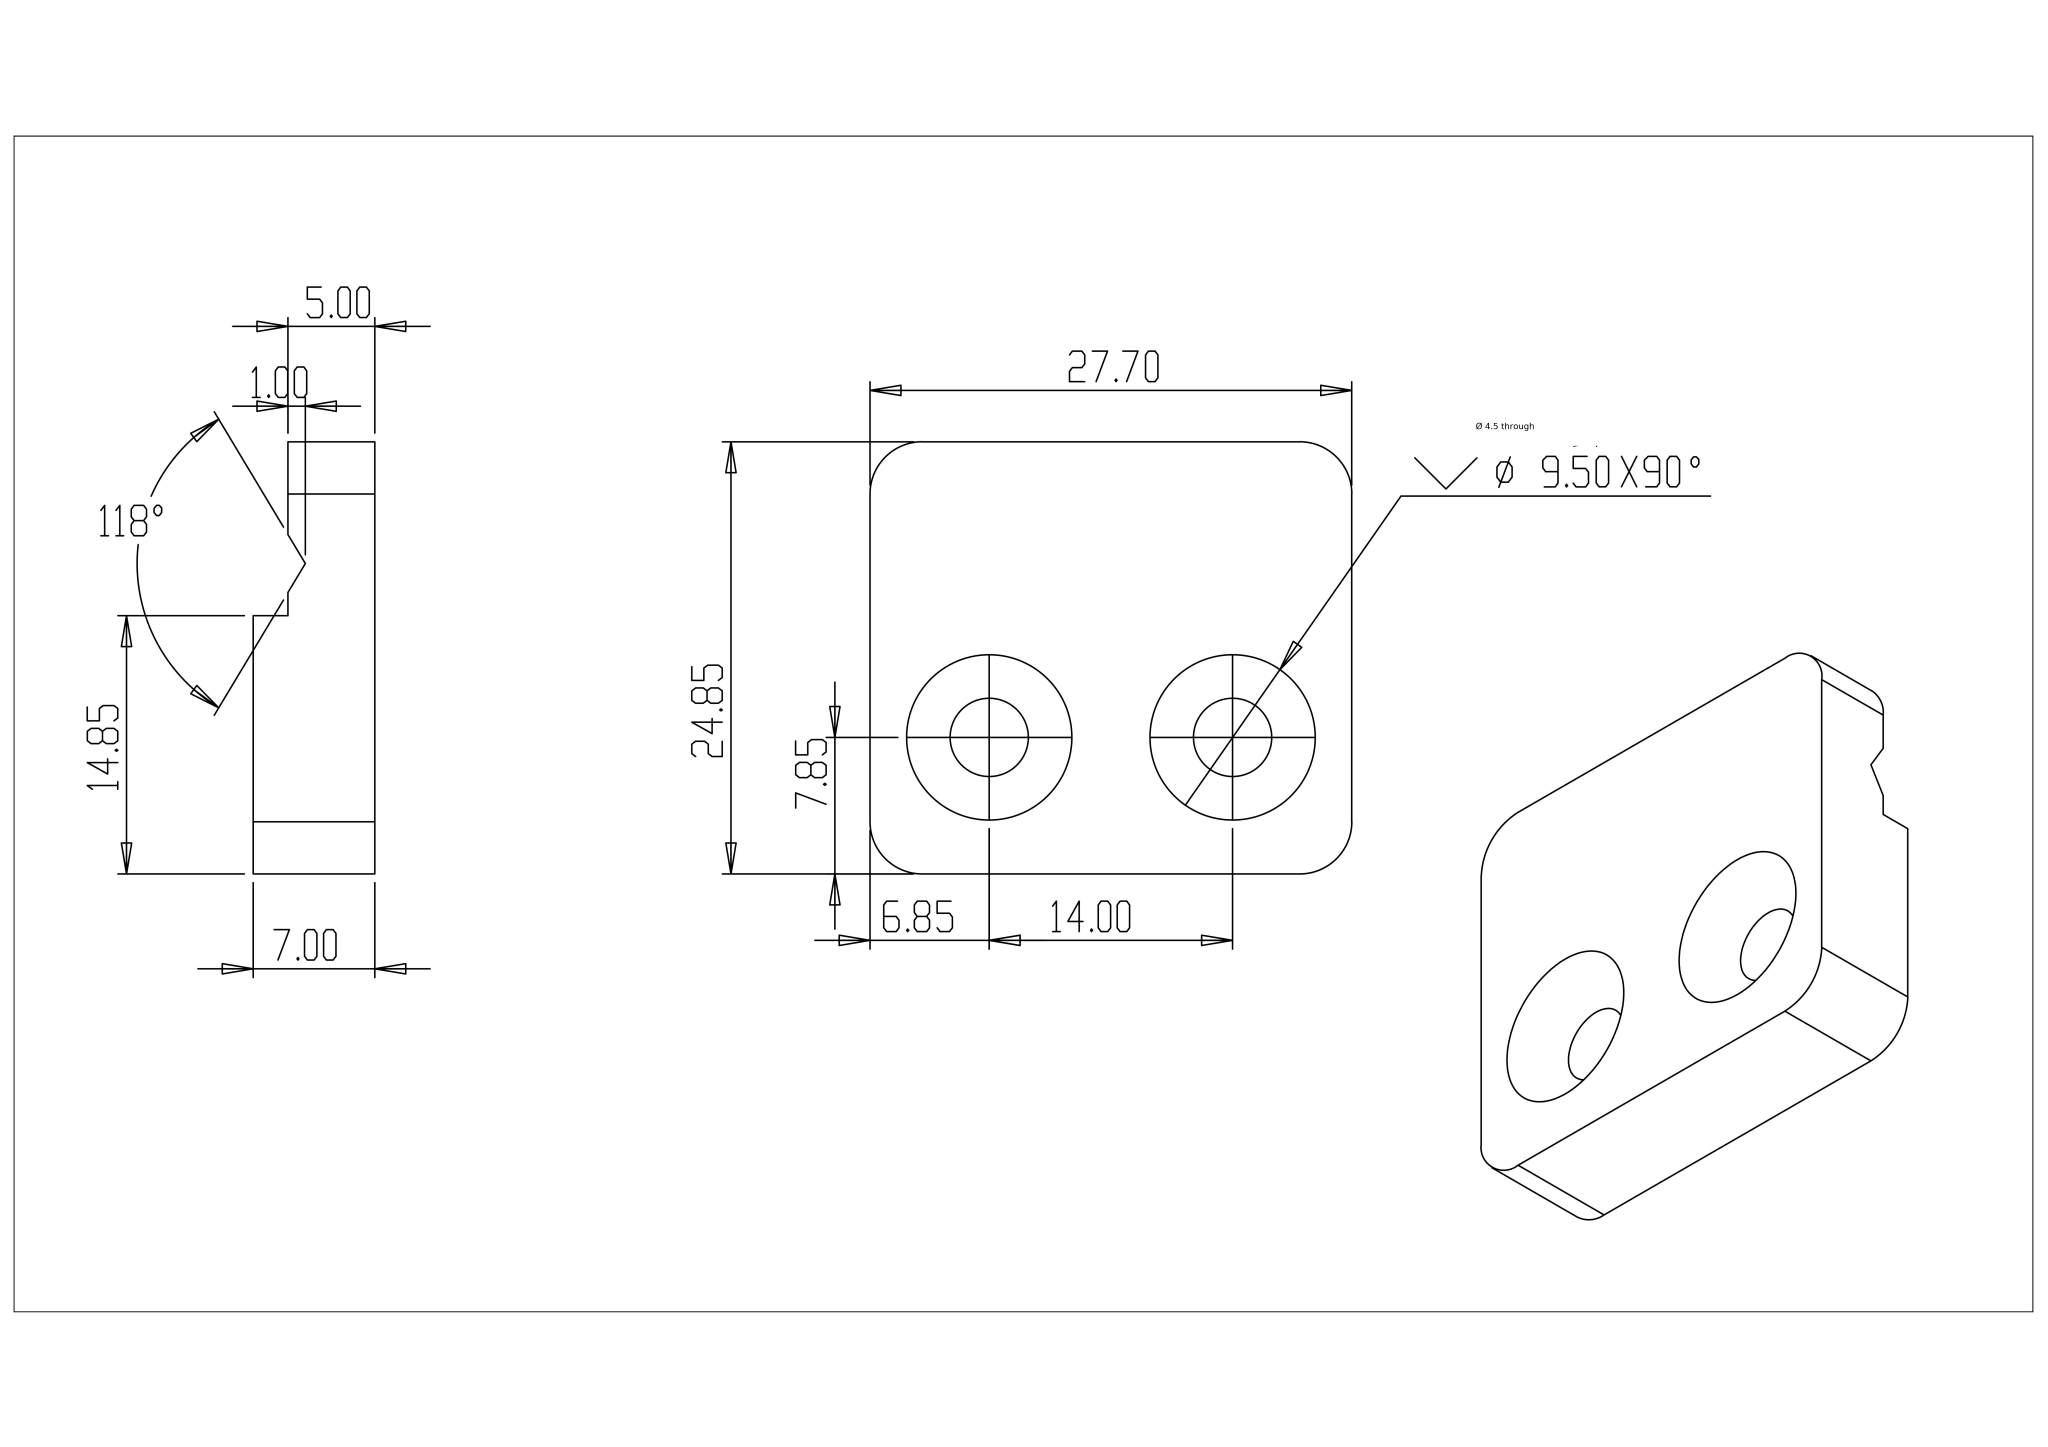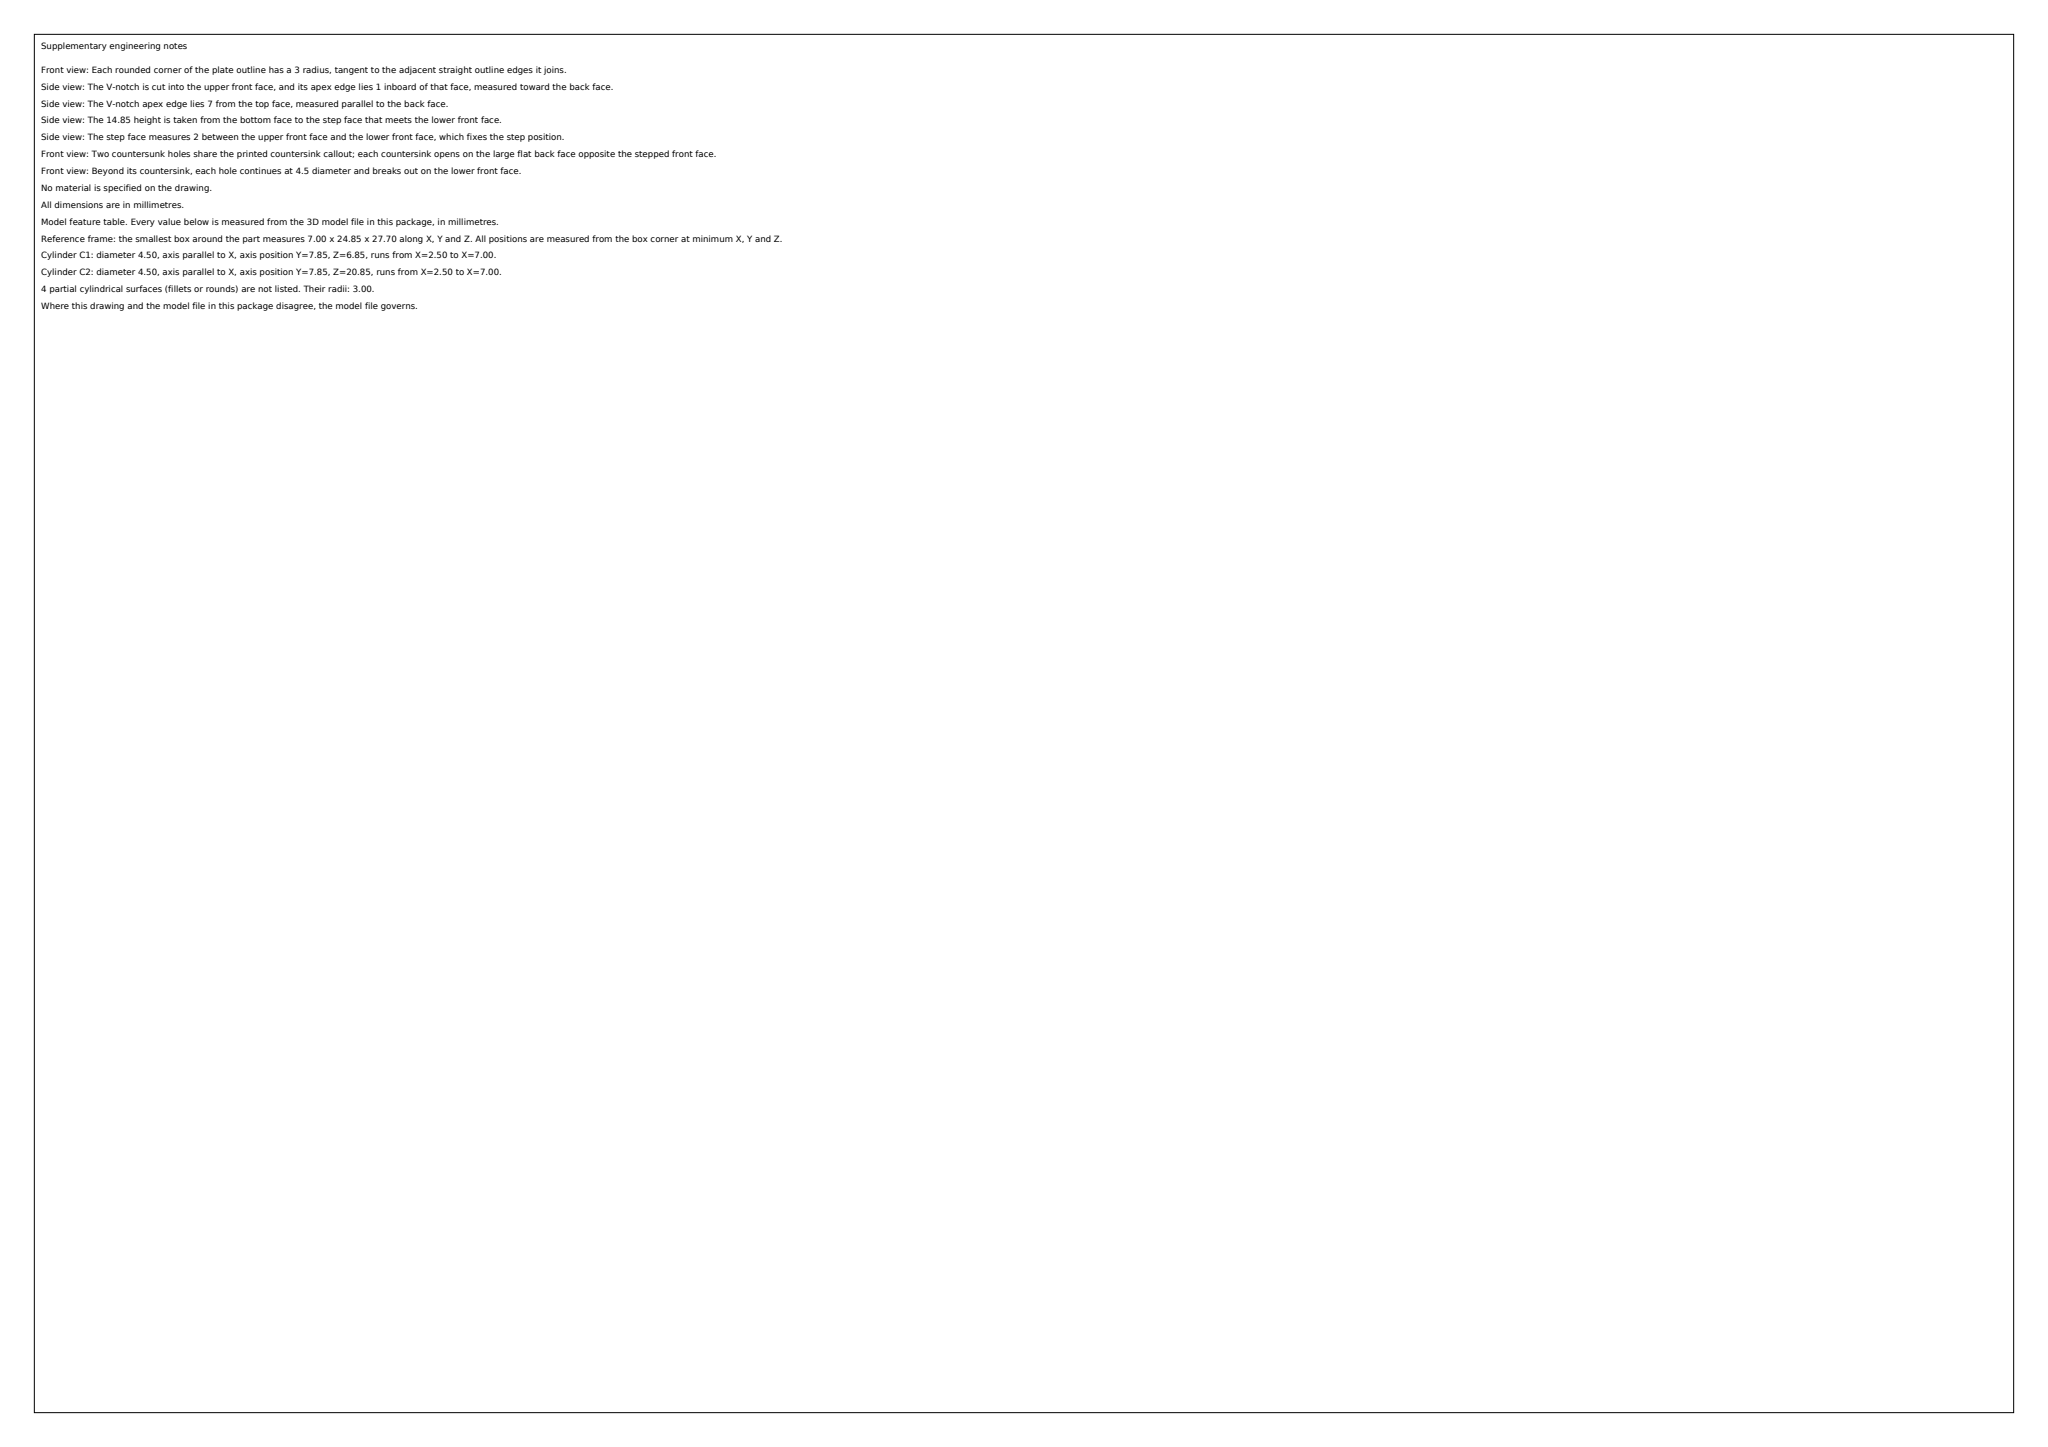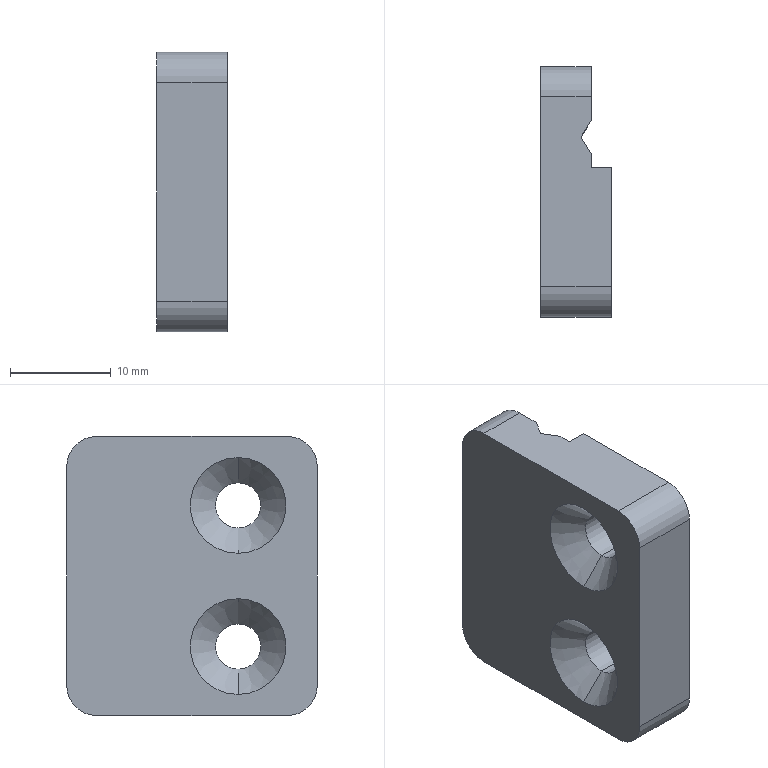Part | SolidWorks | mm | 1 solid | 23 faces | box 7 x 24.85 x 27.7 mm | volume 3828 mm3 | plane 11 | cylinder 8 | cone 4 | commonest cylinder face diameters 4.5 x4 6 x4
Drawing notes:
Ø9.50 X 90° CSK NEAR & FAR SIDE | from the solid: cones[90.0,ref_dia 4.5] count=4 for 2 thru holes -> csk on both x=0 and x=7/5 faces
2X Ø4.5 THRU, CSK Ø9.50 X 90° BOTH SIDES | from the solid: cylinders dia 4.5 at (y7.85,z6.85) and (y7.85,z20.85), 4 cones total
UNLESS OTHERWISE SPECIFIED ALL DIMS IN MM | from the solid: bbox_xyz 7.0 x 24.85 x 27.7 mm
SIDE VIEW: DEL 1.00; BACK STEP 2.00 DP X 10.00 FROM TOP EDGE | from the solid: x planes 0/5/7: 5.0 thk for y 14.85-24.85 (10.00 wide), 7.0 thk below; no face at 1.00
SIDE VIEW: DEL 118°; STEP FACES SQUARE, NO ANGLED FACE | from the solid: axis_planes only normals x,y,z (x=0,5,7; y=0,14.85,24.85; z=0,27.7); no inclined plane
build123d program:
from build123d import *

# Parameters (mm, degrees)
BOSS_EXTRUDE1_DEPTH = 27.7
FILLET1_R           = 3
CUT_EXTRUDE1_REACH  = 39.866
CHAMFER1_SIZE       = 2.5


with BuildPart() as part:
    # Sketch1 → Boss-Extrude1 (new body)
    with BuildSketch(Plane.XY):
        Polygon((0, -22), (0, -24.85), (7, -24.85), (7, -22), (7, -10), (5.3, -10), (5, -10), (5, -8.667), (4, -7), (5, -5.333), (5, -4.5), (5, -3), (5, 0), (0, 0), (0, -3), align=None)
    extrude(amount=BOSS_EXTRUDE1_DEPTH)

    # Fillet1
    fillet1_edges = [part.edges().sort_by_distance(p)[0] for p in [
        (3.5, -24.85, 27.7),
        (2.5, 0, 0),
        (3.5, -24.85, 0),
        (2.5, 0, 27.7),
    ]]
    fillet(fillet1_edges, radius=FILLET1_R)

    # Sketch2 → Cut-Extrude1 (cut, up to next)
    with BuildSketch(Plane(origin=(7, 0, 0), x_dir=(0, 0, -1), z_dir=(1, 0, 0)), mode=Mode.PRIVATE) as cut_extrude1_sk1:
        with BuildLine():
            ThreePointArc((-9.1, -17), (-6.85, -19.25), (-4.6, -17))
            ThreePointArc((-4.6, -17), (-6.85, -14.75), (-9.1, -17))
        make_face()
    cut_extrude1_tool1 = extrude(cut_extrude1_sk1.sketch, amount=-CUT_EXTRUDE1_REACH, mode=Mode.PRIVATE) & part.part
    # Sketch2 → Cut-Extrude1 (cut, up to next)
    with BuildSketch(Plane(origin=(7, 0, 0), x_dir=(0, 0, -1), z_dir=(1, 0, 0)), mode=Mode.PRIVATE) as cut_extrude1_sk2:
        with BuildLine():
            ThreePointArc((-23.1, -17), (-20.85, -19.25), (-18.6, -17))
            ThreePointArc((-18.6, -17), (-20.85, -14.75), (-23.1, -17))
        make_face()
    cut_extrude1_tool2 = extrude(cut_extrude1_sk2.sketch, amount=-CUT_EXTRUDE1_REACH, mode=Mode.PRIVATE) & part.part
    add(cut_extrude1_tool1.solids().sort_by_distance((7, -17, 6.85))[0], mode=Mode.SUBTRACT)
    add(cut_extrude1_tool2.solids().sort_by_distance((7, -17, 20.85))[0], mode=Mode.SUBTRACT)

    # Chamfer1
    chamfer1_edges = [part.edges().sort_by_distance(p)[0] for p in [
        (0, -17, 9.1),
        (0, -17, 18.6),
    ]]
    chamfer(chamfer1_edges, length=CHAMFER1_SIZE)


solid = part.part
STEP:
#1=CARTESIAN_POINT('',(2.5,-17.,4.6));
#2=VERTEX_POINT('',#1);
#3=CARTESIAN_POINT('',(2.5,-17.,9.1));
#4=VERTEX_POINT('',#3);
#5=CARTESIAN_POINT('',(2.5,-17.,6.85));
#6=DIRECTION('',(-1.,0.,0.));
#7=DIRECTION('',(0.,0.,-1.));
#8=AXIS2_PLACEMENT_3D('',#5,#6,#7);
#9=CIRCLE('',#8,2.25);
#10=EDGE_CURVE('',#2,#4,#9,.T.);
#11=ORIENTED_EDGE('',*,*,#10,.F.);
#12=CARTESIAN_POINT('',(0.,-17.,2.1));
#13=VERTEX_POINT('',#12);
#14=CARTESIAN_POINT('',(2.5,-17.,4.6));
#15=DIRECTION('',(-0.7071,0.,-0.7071));
#16=VECTOR('',#15,1000.);
#17=LINE('',#14,#16);
#18=EDGE_CURVE('',#2,#13,#17,.T.);
#19=ORIENTED_EDGE('',*,*,#18,.T.);
#20=CARTESIAN_POINT('',(0.,-17.,11.6));
#21=VERTEX_POINT('',#20);
#22=CARTESIAN_POINT('',(0.,-17.,6.85));
#23=DIRECTION('',(1.,0.,0.));
#24=DIRECTION('',(0.,0.,-1.));
#25=AXIS2_PLACEMENT_3D('',#22,#23,#24);
#26=CIRCLE('',#25,4.75);
#27=EDGE_CURVE('',#21,#13,#26,.T.);
#28=ORIENTED_EDGE('',*,*,#27,.F.);
#29=CARTESIAN_POINT('',(2.5,-17.,9.1));
#30=DIRECTION('',(-0.7071,0.,0.7071));
#31=VECTOR('',#30,1000.);
#32=LINE('',#29,#31);
#33=EDGE_CURVE('',#4,#21,#32,.T.);
#34=ORIENTED_EDGE('',*,*,#33,.F.);
#35=EDGE_LOOP('',(#11,#19,#28,#34));
#36=FACE_OUTER_BOUND('',#35,.T.);
#37=CARTESIAN_POINT('',(2.5,-17.,6.85));
#38=DIRECTION('',(-1.,0.,0.));
#39=DIRECTION('',(0.,0.,1.));
#40=AXIS2_PLACEMENT_3D('',#37,#38,#39);
#41=CONICAL_SURFACE('',#40,2.25,0.7854);
#42=ADVANCED_FACE('',(#36),#41,.F.);
#43=CARTESIAN_POINT('',(2.5,-17.,18.6));
#44=VERTEX_POINT('',#43);
#45=CARTESIAN_POINT('',(2.5,-17.,23.1));
#46=VERTEX_POINT('',#45);
#47=CARTESIAN_POINT('',(2.5,-17.,20.85));
#48=DIRECTION('',(-1.,0.,0.));
#49=DIRECTION('',(0.,0.,-1.));
#50=AXIS2_PLACEMENT_3D('',#47,#48,#49);
#51=CIRCLE('',#50,2.25);
#52=EDGE_CURVE('',#44,#46,#51,.T.);
#53=ORIENTED_EDGE('',*,*,#52,.F.);
#54=CARTESIAN_POINT('',(0.,-17.,16.1));
#55=VERTEX_POINT('',#54);
#56=CARTESIAN_POINT('',(2.5,-17.,18.6));
#57=DIRECTION('',(-0.7071,0.,-0.7071));
#58=VECTOR('',#57,1000.);
#59=LINE('',#56,#58);
#60=EDGE_CURVE('',#44,#55,#59,.T.);
#61=ORIENTED_EDGE('',*,*,#60,.T.);
#62=CARTESIAN_POINT('',(0.,-17.,25.6));
#63=VERTEX_POINT('',#62);
#64=CARTESIAN_POINT('',(0.,-17.,20.85));
#65=DIRECTION('',(1.,0.,0.));
#66=DIRECTION('',(0.,0.,-1.));
#67=AXIS2_PLACEMENT_3D('',#64,#65,#66);
#68=CIRCLE('',#67,4.75);
#69=EDGE_CURVE('',#63,#55,#68,.T.);
#70=ORIENTED_EDGE('',*,*,#69,.F.);
#71=CARTESIAN_POINT('',(2.5,-17.,23.1));
#72=DIRECTION('',(-0.7071,0.,0.7071));
#73=VECTOR('',#72,1000.);
#74=LINE('',#71,#73);
#75=EDGE_CURVE('',#46,#63,#74,.T.);
#76=ORIENTED_EDGE('',*,*,#75,.F.);
#77=EDGE_LOOP('',(#53,#61,#70,#76));
#78=FACE_OUTER_BOUND('',#77,.T.);
#79=CARTESIAN_POINT('',(2.5,-17.,20.85));
#80=DIRECTION('',(-1.,0.,0.));
#81=DIRECTION('',(0.,0.,1.));
#82=AXIS2_PLACEMENT_3D('',#79,#80,#81);
#83=CONICAL_SURFACE('',#82,2.25,0.7854);
#84=ADVANCED_FACE('',(#78),#83,.F.);
#85=ORIENTED_EDGE('',*,*,#10,.T.);
#86=CARTESIAN_POINT('',(7.,-17.,9.1));
#87=VERTEX_POINT('',#86);
#88=CARTESIAN_POINT('',(-0.001,-17.,9.1));
#89=DIRECTION('',(1.,0.,0.));
#90=VECTOR('',#89,1000.);
#91=LINE('',#88,#90);
#92=EDGE_CURVE('',#4,#87,#91,.T.);
#93=ORIENTED_EDGE('',*,*,#92,.T.);
#94=CARTESIAN_POINT('',(7.,-17.,4.6));
#95=VERTEX_POINT('',#94);
#96=CARTESIAN_POINT('',(7.,-17.,6.85));
#97=DIRECTION('',(1.,0.,0.));
#98=DIRECTION('',(0.,0.,-1.));
#99=AXIS2_PLACEMENT_3D('',#96,#97,#98);
#100=CIRCLE('',#99,2.25);
#101=EDGE_CURVE('',#87,#95,#100,.T.);
#102=ORIENTED_EDGE('',*,*,#101,.T.);
#103=CARTESIAN_POINT('',(-0.001,-17.,4.6));
#104=DIRECTION('',(1.,0.,0.));
#105=VECTOR('',#104,1000.);
#106=LINE('',#103,#105);
#107=EDGE_CURVE('',#2,#95,#106,.T.);
#108=ORIENTED_EDGE('',*,*,#107,.F.);
#109=EDGE_LOOP('',(#85,#93,#102,#108));
#110=FACE_OUTER_BOUND('',#109,.T.);
#111=CARTESIAN_POINT('',(-0.001,-17.,6.85));
#112=DIRECTION('',(1.,0.,0.));
#113=DIRECTION('',(0.,0.,-1.));
#114=AXIS2_PLACEMENT_3D('',#111,#112,#113);
#115=CYLINDRICAL_SURFACE('',#114,2.25);
#116=ADVANCED_FACE('',(#110),#115,.F.);
#117=ORIENTED_EDGE('',*,*,#52,.T.);
#118=CARTESIAN_POINT('',(7.,-17.,23.1));
#119=VERTEX_POINT('',#118);
#120=CARTESIAN_POINT('',(-0.001,-17.,23.1));
#121=DIRECTION('',(1.,0.,0.));
#122=VECTOR('',#121,1000.);
#123=LINE('',#120,#122);
#124=EDGE_CURVE('',#46,#119,#123,.T.);
#125=ORIENTED_EDGE('',*,*,#124,.T.);
#126=CARTESIAN_POINT('',(7.,-17.,18.6));
#127=VERTEX_POINT('',#126);
#128=CARTESIAN_POINT('',(7.,-17.,20.85));
#129=DIRECTION('',(1.,0.,0.));
#130=DIRECTION('',(0.,0.,-1.));
#131=AXIS2_PLACEMENT_3D('',#128,#129,#130);
#132=CIRCLE('',#131,2.25);
#133=EDGE_CURVE('',#119,#127,#132,.T.);
#134=ORIENTED_EDGE('',*,*,#133,.T.);
#135=CARTESIAN_POINT('',(-0.001,-17.,18.6));
#136=DIRECTION('',(1.,0.,0.));
#137=VECTOR('',#136,1000.);
#138=LINE('',#135,#137);
#139=EDGE_CURVE('',#44,#127,#138,.T.);
#140=ORIENTED_EDGE('',*,*,#139,.F.);
#141=EDGE_LOOP('',(#117,#125,#134,#140));
#142=FACE_OUTER_BOUND('',#141,.T.);
#143=CARTESIAN_POINT('',(-0.001,-17.,20.85));
#144=DIRECTION('',(1.,0.,0.));
#145=DIRECTION('',(0.,0.,-1.));
#146=AXIS2_PLACEMENT_3D('',#143,#144,#145);
#147=CYLINDRICAL_SURFACE('',#146,2.25);
#148=ADVANCED_FACE('',(#142),#147,.F.);
#149=CARTESIAN_POINT('',(0.,-24.85,24.7));
#150=VERTEX_POINT('',#149);
#151=CARTESIAN_POINT('',(0.,-24.85,3.));
#152=VERTEX_POINT('',#151);
#153=CARTESIAN_POINT('',(0.,-24.85,27.7));
#154=DIRECTION('',(0.,0.,-1.));
#155=VECTOR('',#154,1000.);
#156=LINE('',#153,#155);
#157=EDGE_CURVE('',#150,#152,#156,.T.);
#158=ORIENTED_EDGE('',*,*,#157,.T.);
#159=CARTESIAN_POINT('',(7.,-24.85,3.));
#160=VERTEX_POINT('',#159);
#161=CARTESIAN_POINT('',(0.,-24.85,3.));
#162=DIRECTION('',(1.,0.,0.));
#163=VECTOR('',#162,1000.);
#164=LINE('',#161,#163);
#165=EDGE_CURVE('',#152,#160,#164,.T.);
#166=ORIENTED_EDGE('',*,*,#165,.T.);
#167=CARTESIAN_POINT('',(7.,-24.85,24.7));
#168=VERTEX_POINT('',#167);
#169=CARTESIAN_POINT('',(7.,-24.85,27.7));
#170=DIRECTION('',(0.,0.,-1.));
#171=VECTOR('',#170,1000.);
#172=LINE('',#169,#171);
#173=EDGE_CURVE('',#168,#160,#172,.T.);
#174=ORIENTED_EDGE('',*,*,#173,.F.);
#175=CARTESIAN_POINT('',(0.,-24.85,24.7));
#176=DIRECTION('',(-1.,0.,0.));
#177=VECTOR('',#176,1000.);
#178=LINE('',#175,#177);
#179=EDGE_CURVE('',#168,#150,#178,.T.);
#180=ORIENTED_EDGE('',*,*,#179,.T.);
#181=EDGE_LOOP('',(#158,#166,#174,#180));
#182=FACE_OUTER_BOUND('',#181,.T.);
#183=CARTESIAN_POINT('',(0.,-24.85,27.7));
#184=DIRECTION('',(0.,1.,0.));
#185=DIRECTION('',(0.,0.,1.));
#186=AXIS2_PLACEMENT_3D('',#183,#184,#185);
#187=PLANE('',#186);
#188=ADVANCED_FACE('',(#182),#187,.F.);
#189=CARTESIAN_POINT('',(7.,-17.,6.85));
#190=DIRECTION('',(1.,0.,0.));
#191=DIRECTION('',(0.,0.,-1.));
#192=AXIS2_PLACEMENT_3D('',#189,#190,#191);
#193=CIRCLE('',#192,2.25);
#194=EDGE_CURVE('',#95,#87,#193,.T.);
#195=ORIENTED_EDGE('',*,*,#194,.F.);
#196=ORIENTED_EDGE('',*,*,#101,.F.);
#197=EDGE_LOOP('',(#195,#196));
#198=FACE_BOUND('',#197,.T.);
#199=CARTESIAN_POINT('',(7.,-17.,20.85));
#200=DIRECTION('',(1.,0.,0.));
#201=DIRECTION('',(0.,0.,-1.));
#202=AXIS2_PLACEMENT_3D('',#199,#200,#201);
#203=CIRCLE('',#202,2.25);
#204=EDGE_CURVE('',#127,#119,#203,.T.);
#205=ORIENTED_EDGE('',*,*,#204,.F.);
#206=ORIENTED_EDGE('',*,*,#133,.F.);
#207=EDGE_LOOP('',(#205,#206));
#208=FACE_BOUND('',#207,.T.);
#209=ORIENTED_EDGE('',*,*,#173,.T.);
#210=CARTESIAN_POINT('',(7.,-21.85,0.));
#211=VERTEX_POINT('',#210);
#212=CARTESIAN_POINT('',(7.,-21.85,3.));
#213=DIRECTION('',(1.,0.,0.));
#214=DIRECTION('',(0.,0.,1.));
#215=AXIS2_PLACEMENT_3D('',#212,#213,#214);
#216=CIRCLE('',#215,3.);
#217=EDGE_CURVE('',#160,#211,#216,.T.);
#218=ORIENTED_EDGE('',*,*,#217,.T.);
#219=CARTESIAN_POINT('',(7.,-10.,0.));
#220=VERTEX_POINT('',#219);
#221=CARTESIAN_POINT('',(7.,-22.,0.));
#222=DIRECTION('',(0.,1.,0.));
#223=VECTOR('',#222,1000.);
#224=LINE('',#221,#223);
#225=EDGE_CURVE('',#211,#220,#224,.T.);
#226=ORIENTED_EDGE('',*,*,#225,.T.);
#227=CARTESIAN_POINT('',(7.,-10.,27.7));
#228=VERTEX_POINT('',#227);
#229=CARTESIAN_POINT('',(7.,-10.,27.7));
#230=DIRECTION('',(0.,0.,-1.));
#231=VECTOR('',#230,1000.);
#232=LINE('',#229,#231);
#233=EDGE_CURVE('',#228,#220,#232,.T.);
#234=ORIENTED_EDGE('',*,*,#233,.F.);
#235=CARTESIAN_POINT('',(7.,-21.85,27.7));
#236=VERTEX_POINT('',#235);
#237=CARTESIAN_POINT('',(7.,-24.85,27.7));
#238=DIRECTION('',(0.,1.,0.));
#239=VECTOR('',#238,1000.);
#240=LINE('',#237,#239);
#241=EDGE_CURVE('',#236,#228,#240,.T.);
#242=ORIENTED_EDGE('',*,*,#241,.F.);
#243=CARTESIAN_POINT('',(7.,-21.85,24.7));
#244=DIRECTION('',(1.,0.,0.));
#245=DIRECTION('',(0.,0.,1.));
#246=AXIS2_PLACEMENT_3D('',#243,#244,#245);
#247=CIRCLE('',#246,3.);
#248=EDGE_CURVE('',#236,#168,#247,.T.);
#249=ORIENTED_EDGE('',*,*,#248,.T.);
#250=EDGE_LOOP('',(#209,#218,#226,#234,#242,#249));
#251=FACE_OUTER_BOUND('',#250,.T.);
#252=CARTESIAN_POINT('',(7.,-22.,27.7));
#253=DIRECTION('',(-1.,0.,0.));
#254=DIRECTION('',(0.,0.,1.));
#255=AXIS2_PLACEMENT_3D('',#252,#253,#254);
#256=PLANE('',#255);
#257=ADVANCED_FACE('',(#198,#208,#251),#256,.F.);
#258=CARTESIAN_POINT('',(5.,-10.,0.));
#259=VERTEX_POINT('',#258);
#260=CARTESIAN_POINT('',(5.,-10.,0.));
#261=DIRECTION('',(-1.,0.,0.));
#262=VECTOR('',#261,1000.);
#263=LINE('',#260,#262);
#264=EDGE_CURVE('',#220,#259,#263,.T.);
#265=ORIENTED_EDGE('',*,*,#264,.T.);
#266=CARTESIAN_POINT('',(5.,-10.,27.7));
#267=VERTEX_POINT('',#266);
#268=CARTESIAN_POINT('',(5.,-10.,27.7));
#269=DIRECTION('',(0.,0.,-1.));
#270=VECTOR('',#269,1000.);
#271=LINE('',#268,#270);
#272=EDGE_CURVE('',#267,#259,#271,.T.);
#273=ORIENTED_EDGE('',*,*,#272,.F.);
#274=CARTESIAN_POINT('',(7.,-10.,27.7));
#275=DIRECTION('',(-1.,0.,0.));
#276=VECTOR('',#275,1000.);
#277=LINE('',#274,#276);
#278=EDGE_CURVE('',#228,#267,#277,.T.);
#279=ORIENTED_EDGE('',*,*,#278,.F.);
#280=ORIENTED_EDGE('',*,*,#233,.T.);
#281=EDGE_LOOP('',(#265,#273,#279,#280));
#282=FACE_OUTER_BOUND('',#281,.T.);
#283=CARTESIAN_POINT('',(5.,-10.,27.7));
#284=DIRECTION('',(0.,-1.,0.));
#285=DIRECTION('',(0.,0.,-1.));
#286=AXIS2_PLACEMENT_3D('',#283,#284,#285);
#287=PLANE('',#286);
#288=ADVANCED_FACE('',(#282),#287,.F.);
#289=CARTESIAN_POINT('',(5.,-8.667,0.));
#290=VERTEX_POINT('',#289);
#291=CARTESIAN_POINT('',(5.,-8.667,0.));
#292=DIRECTION('',(0.,1.,0.));
#293=VECTOR('',#292,1000.);
#294=LINE('',#291,#293);
#295=EDGE_CURVE('',#259,#290,#294,.T.);
#296=ORIENTED_EDGE('',*,*,#295,.T.);
#297=CARTESIAN_POINT('',(5.,-8.667,27.7));
#298=VERTEX_POINT('',#297);
#299=CARTESIAN_POINT('',(5.,-8.667,27.7));
#300=DIRECTION('',(0.,0.,-1.));
#301=VECTOR('',#300,1000.);
#302=LINE('',#299,#301);
#303=EDGE_CURVE('',#298,#290,#302,.T.);
#304=ORIENTED_EDGE('',*,*,#303,.F.);
#305=CARTESIAN_POINT('',(5.,-8.667,27.7));
#306=DIRECTION('',(0.,1.,0.));
#307=VECTOR('',#306,1000.);
#308=LINE('',#305,#307);
#309=EDGE_CURVE('',#267,#298,#308,.T.);
#310=ORIENTED_EDGE('',*,*,#309,.F.);
#311=ORIENTED_EDGE('',*,*,#272,.T.);
#312=EDGE_LOOP('',(#296,#304,#310,#311));
#313=FACE_OUTER_BOUND('',#312,.T.);
#314=CARTESIAN_POINT('',(5.,-8.667,27.7));
#315=DIRECTION('',(-1.,0.,0.));
#316=DIRECTION('',(-0.,-1.,0.));
#317=AXIS2_PLACEMENT_3D('',#314,#315,#316);
#318=PLANE('',#317);
#319=ADVANCED_FACE('',(#313),#318,.F.);
#320=CARTESIAN_POINT('',(4.,-7.,0.));
#321=VERTEX_POINT('',#320);
#322=CARTESIAN_POINT('',(5.,-8.667,0.));
#323=DIRECTION('',(-0.5145,0.8575,0.));
#324=VECTOR('',#323,1000.);
#325=LINE('',#322,#324);
#326=EDGE_CURVE('',#290,#321,#325,.T.);
#327=ORIENTED_EDGE('',*,*,#326,.T.);
#328=CARTESIAN_POINT('',(4.,-7.,27.7));
#329=VERTEX_POINT('',#328);
#330=CARTESIAN_POINT('',(4.,-7.,27.7));
#331=DIRECTION('',(0.,0.,-1.));
#332=VECTOR('',#331,1000.);
#333=LINE('',#330,#332);
#334=EDGE_CURVE('',#329,#321,#333,.T.);
#335=ORIENTED_EDGE('',*,*,#334,.F.);
#336=CARTESIAN_POINT('',(5.,-8.667,27.7));
#337=DIRECTION('',(-0.5145,0.8575,0.));
#338=VECTOR('',#337,1000.);
#339=LINE('',#336,#338);
#340=EDGE_CURVE('',#298,#329,#339,.T.);
#341=ORIENTED_EDGE('',*,*,#340,.F.);
#342=ORIENTED_EDGE('',*,*,#303,.T.);
#343=EDGE_LOOP('',(#327,#335,#341,#342));
#344=FACE_OUTER_BOUND('',#343,.T.);
#345=CARTESIAN_POINT('',(5.,-8.667,27.7));
#346=DIRECTION('',(-0.8575,-0.5145,0.));
#347=DIRECTION('',(0.5145,-0.8575,0.));
#348=AXIS2_PLACEMENT_3D('',#345,#346,#347);
#349=PLANE('',#348);
#350=ADVANCED_FACE('',(#344),#349,.F.);
#351=CARTESIAN_POINT('',(5.,-5.333,0.));
#352=VERTEX_POINT('',#351);
#353=CARTESIAN_POINT('',(4.,-7.,0.));
#354=DIRECTION('',(0.5145,0.8575,0.));
#355=VECTOR('',#354,1000.);
#356=LINE('',#353,#355);
#357=EDGE_CURVE('',#321,#352,#356,.T.);
#358=ORIENTED_EDGE('',*,*,#357,.T.);
#359=CARTESIAN_POINT('',(5.,-5.333,27.7));
#360=VERTEX_POINT('',#359);
#361=CARTESIAN_POINT('',(5.,-5.333,27.7));
#362=DIRECTION('',(0.,0.,-1.));
#363=VECTOR('',#362,1000.);
#364=LINE('',#361,#363);
#365=EDGE_CURVE('',#360,#352,#364,.T.);
#366=ORIENTED_EDGE('',*,*,#365,.F.);
#367=CARTESIAN_POINT('',(4.,-7.,27.7));
#368=DIRECTION('',(0.5145,0.8575,0.));
#369=VECTOR('',#368,1000.);
#370=LINE('',#367,#369);
#371=EDGE_CURVE('',#329,#360,#370,.T.);
#372=ORIENTED_EDGE('',*,*,#371,.F.);
#373=ORIENTED_EDGE('',*,*,#334,.T.);
#374=EDGE_LOOP('',(#358,#366,#372,#373));
#375=FACE_OUTER_BOUND('',#374,.T.);
#376=CARTESIAN_POINT('',(4.,-7.,27.7));
#377=DIRECTION('',(-0.8575,0.5145,0.));
#378=DIRECTION('',(-0.5145,-0.8575,0.));
#379=AXIS2_PLACEMENT_3D('',#376,#377,#378);
#380=PLANE('',#379);
#381=ADVANCED_FACE('',(#375),#380,.F.);
#382=CARTESIAN_POINT('',(5.,-3.,0.));
#383=VERTEX_POINT('',#382);
#384=CARTESIAN_POINT('',(5.,-3.,0.));
#385=DIRECTION('',(0.,1.,0.));
#386=VECTOR('',#385,1000.);
#387=LINE('',#384,#386);
#388=EDGE_CURVE('',#352,#383,#387,.T.);
#389=ORIENTED_EDGE('',*,*,#388,.T.);
#390=CARTESIAN_POINT('',(5.,0.,3.));
#391=VERTEX_POINT('',#390);
#392=CARTESIAN_POINT('',(5.,-3.,3.));
#393=DIRECTION('',(1.,0.,0.));
#394=DIRECTION('',(0.,0.,1.));
#395=AXIS2_PLACEMENT_3D('',#392,#393,#394);
#396=CIRCLE('',#395,3.);
#397=EDGE_CURVE('',#383,#391,#396,.T.);
#398=ORIENTED_EDGE('',*,*,#397,.T.);
#399=CARTESIAN_POINT('',(5.,0.,24.7));
#400=VERTEX_POINT('',#399);
#401=CARTESIAN_POINT('',(5.,0.,27.7));
#402=DIRECTION('',(0.,0.,-1.));
#403=VECTOR('',#402,1000.);
#404=LINE('',#401,#403);
#405=EDGE_CURVE('',#400,#391,#404,.T.);
#406=ORIENTED_EDGE('',*,*,#405,.F.);
#407=CARTESIAN_POINT('',(5.,-3.,27.7));
#408=VERTEX_POINT('',#407);
#409=CARTESIAN_POINT('',(5.,-3.,24.7));
#410=DIRECTION('',(1.,0.,0.));
#411=DIRECTION('',(0.,0.,1.));
#412=AXIS2_PLACEMENT_3D('',#409,#410,#411);
#413=CIRCLE('',#412,3.);
#414=EDGE_CURVE('',#400,#408,#413,.T.);
#415=ORIENTED_EDGE('',*,*,#414,.T.);
#416=CARTESIAN_POINT('',(5.,-4.5,27.7));
#417=DIRECTION('',(0.,1.,0.));
#418=VECTOR('',#417,1000.);
#419=LINE('',#416,#418);
#420=EDGE_CURVE('',#360,#408,#419,.T.);
#421=ORIENTED_EDGE('',*,*,#420,.F.);
#422=ORIENTED_EDGE('',*,*,#365,.T.);
#423=EDGE_LOOP('',(#389,#398,#406,#415,#421,#422));
#424=FACE_OUTER_BOUND('',#423,.T.);
#425=CARTESIAN_POINT('',(5.,-3.,27.7));
#426=DIRECTION('',(-1.,0.,0.));
#427=DIRECTION('',(0.,0.,1.));
#428=AXIS2_PLACEMENT_3D('',#425,#426,#427);
#429=PLANE('',#428);
#430=ADVANCED_FACE('',(#424),#429,.F.);
#431=ORIENTED_EDGE('',*,*,#405,.T.);
#432=CARTESIAN_POINT('',(0.,0.,3.));
#433=VERTEX_POINT('',#432);
#434=CARTESIAN_POINT('',(5.,0.,3.));
#435=DIRECTION('',(-1.,0.,0.));
#436=VECTOR('',#435,1000.);
#437=LINE('',#434,#436);
#438=EDGE_CURVE('',#391,#433,#437,.T.);
#439=ORIENTED_EDGE('',*,*,#438,.T.);
#440=CARTESIAN_POINT('',(0.,0.,24.7));
#441=VERTEX_POINT('',#440);
#442=CARTESIAN_POINT('',(0.,0.,27.7));
#443=DIRECTION('',(0.,0.,-1.));
#444=VECTOR('',#443,1000.);
#445=LINE('',#442,#444);
#446=EDGE_CURVE('',#441,#433,#445,.T.);
#447=ORIENTED_EDGE('',*,*,#446,.F.);
#448=CARTESIAN_POINT('',(5.,0.,24.7));
#449=DIRECTION('',(1.,0.,0.));
#450=VECTOR('',#449,1000.);
#451=LINE('',#448,#450);
#452=EDGE_CURVE('',#441,#400,#451,.T.);
#453=ORIENTED_EDGE('',*,*,#452,.T.);
#454=EDGE_LOOP('',(#431,#439,#447,#453));
#455=FACE_OUTER_BOUND('',#454,.T.);
#456=CARTESIAN_POINT('',(5.,0.,27.7));
#457=DIRECTION('',(0.,-1.,0.));
#458=DIRECTION('',(0.,0.,-1.));
#459=AXIS2_PLACEMENT_3D('',#456,#457,#458);
#460=PLANE('',#459);
#461=ADVANCED_FACE('',(#455),#460,.F.);
#462=ORIENTED_EDGE('',*,*,#69,.T.);
#463=CARTESIAN_POINT('',(0.,-17.,20.85));
#464=DIRECTION('',(1.,0.,0.));
#465=DIRECTION('',(0.,0.,-1.));
#466=AXIS2_PLACEMENT_3D('',#463,#464,#465);
#467=CIRCLE('',#466,4.75);
#468=EDGE_CURVE('',#55,#63,#467,.T.);
#469=ORIENTED_EDGE('',*,*,#468,.T.);
#470=EDGE_LOOP('',(#462,#469));
#471=FACE_BOUND('',#470,.T.);
#472=ORIENTED_EDGE('',*,*,#27,.T.);
#473=CARTESIAN_POINT('',(0.,-17.,6.85));
#474=DIRECTION('',(1.,0.,0.));
#475=DIRECTION('',(0.,0.,-1.));
#476=AXIS2_PLACEMENT_3D('',#473,#474,#475);
#477=CIRCLE('',#476,4.75);
#478=EDGE_CURVE('',#13,#21,#477,.T.);
#479=ORIENTED_EDGE('',*,*,#478,.T.);
#480=EDGE_LOOP('',(#472,#479));
#481=FACE_BOUND('',#480,.T.);
#482=ORIENTED_EDGE('',*,*,#446,.T.);
#483=CARTESIAN_POINT('',(0.,-3.,0.));
#484=VERTEX_POINT('',#483);
#485=CARTESIAN_POINT('',(0.,-3.,3.));
#486=DIRECTION('',(-1.,0.,0.));
#487=DIRECTION('',(0.,0.,-1.));
#488=AXIS2_PLACEMENT_3D('',#485,#486,#487);
#489=CIRCLE('',#488,3.);
#490=EDGE_CURVE('',#433,#484,#489,.T.);
#491=ORIENTED_EDGE('',*,*,#490,.T.);
#492=CARTESIAN_POINT('',(0.,-21.85,0.));
#493=VERTEX_POINT('',#492);
#494=CARTESIAN_POINT('',(0.,0.,0.));
#495=DIRECTION('',(0.,-1.,0.));
#496=VECTOR('',#495,1000.);
#497=LINE('',#494,#496);
#498=EDGE_CURVE('',#484,#493,#497,.T.);
#499=ORIENTED_EDGE('',*,*,#498,.T.);
#500=CARTESIAN_POINT('',(0.,-21.85,3.));
#501=DIRECTION('',(-1.,0.,0.));
#502=DIRECTION('',(0.,0.,-1.));
#503=AXIS2_PLACEMENT_3D('',#500,#501,#502);
#504=CIRCLE('',#503,3.);
#505=EDGE_CURVE('',#493,#152,#504,.T.);
#506=ORIENTED_EDGE('',*,*,#505,.T.);
#507=ORIENTED_EDGE('',*,*,#157,.F.);
#508=CARTESIAN_POINT('',(0.,-21.85,27.7));
#509=VERTEX_POINT('',#508);
#510=CARTESIAN_POINT('',(0.,-21.85,24.7));
#511=DIRECTION('',(-1.,0.,0.));
#512=DIRECTION('',(0.,0.,-1.));
#513=AXIS2_PLACEMENT_3D('',#510,#511,#512);
#514=CIRCLE('',#513,3.);
#515=EDGE_CURVE('',#150,#509,#514,.T.);
#516=ORIENTED_EDGE('',*,*,#515,.T.);
#517=CARTESIAN_POINT('',(0.,-3.,27.7));
#518=VERTEX_POINT('',#517);
#519=CARTESIAN_POINT('',(0.,-3.,27.7));
#520=DIRECTION('',(0.,-1.,0.));
#521=VECTOR('',#520,1000.);
#522=LINE('',#519,#521);
#523=EDGE_CURVE('',#518,#509,#522,.T.);
#524=ORIENTED_EDGE('',*,*,#523,.F.);
#525=CARTESIAN_POINT('',(0.,-3.,24.7));
#526=DIRECTION('',(-1.,0.,0.));
#527=DIRECTION('',(0.,0.,-1.));
#528=AXIS2_PLACEMENT_3D('',#525,#526,#527);
#529=CIRCLE('',#528,3.);
#530=EDGE_CURVE('',#518,#441,#529,.T.);
#531=ORIENTED_EDGE('',*,*,#530,.T.);
#532=EDGE_LOOP('',(#482,#491,#499,#506,#507,#516,#524,#531));
#533=FACE_OUTER_BOUND('',#532,.T.);
#534=CARTESIAN_POINT('',(0.,0.,27.7));
#535=DIRECTION('',(1.,0.,0.));
#536=DIRECTION('',(0.,0.,-1.));
#537=AXIS2_PLACEMENT_3D('',#534,#535,#536);
#538=PLANE('',#537);
#539=ADVANCED_FACE('',(#471,#481,#533),#538,.F.);
#540=ORIENTED_EDGE('',*,*,#420,.T.);
#541=CARTESIAN_POINT('',(0.,-3.,27.7));
#542=DIRECTION('',(-1.,0.,0.));
#543=VECTOR('',#542,1000.);
#544=LINE('',#541,#543);
#545=EDGE_CURVE('',#408,#518,#544,.T.);
#546=ORIENTED_EDGE('',*,*,#545,.T.);
#547=ORIENTED_EDGE('',*,*,#523,.T.);
#548=CARTESIAN_POINT('',(7.,-21.85,27.7));
#549=DIRECTION('',(1.,0.,0.));
#550=VECTOR('',#549,1000.);
#551=LINE('',#548,#550);
#552=EDGE_CURVE('',#509,#236,#551,.T.);
#553=ORIENTED_EDGE('',*,*,#552,.T.);
#554=ORIENTED_EDGE('',*,*,#241,.T.);
#555=ORIENTED_EDGE('',*,*,#278,.T.);
#556=ORIENTED_EDGE('',*,*,#309,.T.);
#557=ORIENTED_EDGE('',*,*,#340,.T.);
#558=ORIENTED_EDGE('',*,*,#371,.T.);
#559=EDGE_LOOP('',(#540,#546,#547,#553,#554,#555,#556,#557,#558));
#560=FACE_OUTER_BOUND('',#559,.T.);
#561=CARTESIAN_POINT('',(0.,0.,27.7));
#562=DIRECTION('',(0.,0.,1.));
#563=DIRECTION('',(1.,0.,0.));
#564=AXIS2_PLACEMENT_3D('',#561,#562,#563);
#565=PLANE('',#564);
#566=ADVANCED_FACE('',(#560),#565,.T.);
#567=ORIENTED_EDGE('',*,*,#498,.F.);
#568=CARTESIAN_POINT('',(0.,-3.,0.));
#569=DIRECTION('',(1.,0.,0.));
#570=VECTOR('',#569,1000.);
#571=LINE('',#568,#570);
#572=EDGE_CURVE('',#484,#383,#571,.T.);
#573=ORIENTED_EDGE('',*,*,#572,.T.);
#574=ORIENTED_EDGE('',*,*,#388,.F.);
#575=ORIENTED_EDGE('',*,*,#357,.F.);
#576=ORIENTED_EDGE('',*,*,#326,.F.);
#577=ORIENTED_EDGE('',*,*,#295,.F.);
#578=ORIENTED_EDGE('',*,*,#264,.F.);
#579=ORIENTED_EDGE('',*,*,#225,.F.);
#580=CARTESIAN_POINT('',(0.,-21.85,0.));
#581=DIRECTION('',(-1.,0.,0.));
#582=VECTOR('',#581,1000.);
#583=LINE('',#580,#582);
#584=EDGE_CURVE('',#211,#493,#583,.T.);
#585=ORIENTED_EDGE('',*,*,#584,.T.);
#586=EDGE_LOOP('',(#567,#573,#574,#575,#576,#577,#578,#579,#585));
#587=FACE_OUTER_BOUND('',#586,.T.);
#588=CARTESIAN_POINT('',(0.,0.,0.));
#589=DIRECTION('',(0.,0.,1.));
#590=DIRECTION('',(1.,0.,0.));
#591=AXIS2_PLACEMENT_3D('',#588,#589,#590);
#592=PLANE('',#591);
#593=ADVANCED_FACE('',(#587),#592,.F.);
#594=ORIENTED_EDGE('',*,*,#397,.F.);
#595=ORIENTED_EDGE('',*,*,#572,.F.);
#596=ORIENTED_EDGE('',*,*,#490,.F.);
#597=ORIENTED_EDGE('',*,*,#438,.F.);
#598=EDGE_LOOP('',(#594,#595,#596,#597));
#599=FACE_OUTER_BOUND('',#598,.T.);
#600=CARTESIAN_POINT('',(5.,-3.,3.));
#601=DIRECTION('',(-1.,0.,0.));
#602=DIRECTION('',(0.,0.,1.));
#603=AXIS2_PLACEMENT_3D('',#600,#601,#602);
#604=CYLINDRICAL_SURFACE('',#603,3.);
#605=ADVANCED_FACE('',(#599),#604,.T.);
#606=ORIENTED_EDGE('',*,*,#414,.F.);
#607=ORIENTED_EDGE('',*,*,#452,.F.);
#608=ORIENTED_EDGE('',*,*,#530,.F.);
#609=ORIENTED_EDGE('',*,*,#545,.F.);
#610=EDGE_LOOP('',(#606,#607,#608,#609));
#611=FACE_OUTER_BOUND('',#610,.T.);
#612=CARTESIAN_POINT('',(0.,-3.,24.7));
#613=DIRECTION('',(1.,0.,0.));
#614=DIRECTION('',(0.,0.,-1.));
#615=AXIS2_PLACEMENT_3D('',#612,#613,#614);
#616=CYLINDRICAL_SURFACE('',#615,3.);
#617=ADVANCED_FACE('',(#611),#616,.T.);
#618=ORIENTED_EDGE('',*,*,#505,.F.);
#619=ORIENTED_EDGE('',*,*,#584,.F.);
#620=ORIENTED_EDGE('',*,*,#217,.F.);
#621=ORIENTED_EDGE('',*,*,#165,.F.);
#622=EDGE_LOOP('',(#618,#619,#620,#621));
#623=FACE_OUTER_BOUND('',#622,.T.);
#624=CARTESIAN_POINT('',(0.,-21.85,3.));
#625=DIRECTION('',(1.,0.,0.));
#626=DIRECTION('',(0.,0.,-1.));
#627=AXIS2_PLACEMENT_3D('',#624,#625,#626);
#628=CYLINDRICAL_SURFACE('',#627,3.);
#629=ADVANCED_FACE('',(#623),#628,.T.);
#630=ORIENTED_EDGE('',*,*,#515,.F.);
#631=ORIENTED_EDGE('',*,*,#179,.F.);
#632=ORIENTED_EDGE('',*,*,#248,.F.);
#633=ORIENTED_EDGE('',*,*,#552,.F.);
#634=EDGE_LOOP('',(#630,#631,#632,#633));
#635=FACE_OUTER_BOUND('',#634,.T.);
#636=CARTESIAN_POINT('',(0.,-21.85,24.7));
#637=DIRECTION('',(-1.,0.,0.));
#638=DIRECTION('',(0.,0.,1.));
#639=AXIS2_PLACEMENT_3D('',#636,#637,#638);
#640=CYLINDRICAL_SURFACE('',#639,3.);
#641=ADVANCED_FACE('',(#635),#640,.T.);
#642=ORIENTED_EDGE('',*,*,#124,.F.);
#643=CARTESIAN_POINT('',(2.5,-17.,20.85));
#644=DIRECTION('',(-1.,0.,0.));
#645=DIRECTION('',(0.,0.,-1.));
#646=AXIS2_PLACEMENT_3D('',#643,#644,#645);
#647=CIRCLE('',#646,2.25);
#648=EDGE_CURVE('',#46,#44,#647,.T.);
#649=ORIENTED_EDGE('',*,*,#648,.T.);
#650=ORIENTED_EDGE('',*,*,#139,.T.);
#651=ORIENTED_EDGE('',*,*,#204,.T.);
#652=EDGE_LOOP('',(#642,#649,#650,#651));
#653=FACE_OUTER_BOUND('',#652,.T.);
#654=CARTESIAN_POINT('',(-0.001,-17.,20.85));
#655=DIRECTION('',(1.,0.,0.));
#656=DIRECTION('',(0.,0.,-1.));
#657=AXIS2_PLACEMENT_3D('',#654,#655,#656);
#658=CYLINDRICAL_SURFACE('',#657,2.25);
#659=ADVANCED_FACE('',(#653),#658,.F.);
#660=ORIENTED_EDGE('',*,*,#92,.F.);
#661=CARTESIAN_POINT('',(2.5,-17.,6.85));
#662=DIRECTION('',(-1.,0.,0.));
#663=DIRECTION('',(0.,0.,-1.));
#664=AXIS2_PLACEMENT_3D('',#661,#662,#663);
#665=CIRCLE('',#664,2.25);
#666=EDGE_CURVE('',#4,#2,#665,.T.);
#667=ORIENTED_EDGE('',*,*,#666,.T.);
#668=ORIENTED_EDGE('',*,*,#107,.T.);
#669=ORIENTED_EDGE('',*,*,#194,.T.);
#670=EDGE_LOOP('',(#660,#667,#668,#669));
#671=FACE_OUTER_BOUND('',#670,.T.);
#672=CARTESIAN_POINT('',(-0.001,-17.,6.85));
#673=DIRECTION('',(1.,0.,0.));
#674=DIRECTION('',(0.,0.,-1.));
#675=AXIS2_PLACEMENT_3D('',#672,#673,#674);
#676=CYLINDRICAL_SURFACE('',#675,2.25);
#677=ADVANCED_FACE('',(#671),#676,.F.);
#678=ORIENTED_EDGE('',*,*,#60,.F.);
#679=ORIENTED_EDGE('',*,*,#648,.F.);
#680=ORIENTED_EDGE('',*,*,#75,.T.);
#681=ORIENTED_EDGE('',*,*,#468,.F.);
#682=EDGE_LOOP('',(#678,#679,#680,#681));
#683=FACE_OUTER_BOUND('',#682,.T.);
#684=CARTESIAN_POINT('',(2.5,-17.,20.85));
#685=DIRECTION('',(-1.,0.,0.));
#686=DIRECTION('',(0.,0.,1.));
#687=AXIS2_PLACEMENT_3D('',#684,#685,#686);
#688=CONICAL_SURFACE('',#687,2.25,0.7854);
#689=ADVANCED_FACE('',(#683),#688,.F.);
#690=ORIENTED_EDGE('',*,*,#18,.F.);
#691=ORIENTED_EDGE('',*,*,#666,.F.);
#692=ORIENTED_EDGE('',*,*,#33,.T.);
#693=ORIENTED_EDGE('',*,*,#478,.F.);
#694=EDGE_LOOP('',(#690,#691,#692,#693));
#695=FACE_OUTER_BOUND('',#694,.T.);
#696=CARTESIAN_POINT('',(2.5,-17.,6.85));
#697=DIRECTION('',(-1.,0.,0.));
#698=DIRECTION('',(0.,0.,1.));
#699=AXIS2_PLACEMENT_3D('',#696,#697,#698);
#700=CONICAL_SURFACE('',#699,2.25,0.7854);
#701=ADVANCED_FACE('',(#695),#700,.F.);
#702=CLOSED_SHELL('',(#42,#84,#116,#148,#188,#257,#288,#319,#350,#381,#430,#461,#539,#566,#593,#605,#617,#629,#641,#659,#677,#689,#701));
#703=MANIFOLD_SOLID_BREP('',#702);
#704=CARTESIAN_POINT('',(0.,0.,0.));
#705=DIRECTION('',(0.,0.,1.));
#706=DIRECTION('',(1.,0.,0.));
#707=AXIS2_PLACEMENT_3D('',#704,#705,#706);
#708=(LENGTH_UNIT()NAMED_UNIT(*)SI_UNIT(.MILLI.,.METRE.));
#709=UNCERTAINTY_MEASURE_WITH_UNIT(LENGTH_MEASURE(0.00001),#708,'','');
#710=(NAMED_UNIT(*)PLANE_ANGLE_UNIT()SI_UNIT($,.RADIAN.));
#711=(NAMED_UNIT(*)SI_UNIT($,.STERADIAN.)SOLID_ANGLE_UNIT());
#712=(GEOMETRIC_REPRESENTATION_CONTEXT(3)GLOBAL_UNCERTAINTY_ASSIGNED_CONTEXT((#709))GLOBAL_UNIT_ASSIGNED_CONTEXT((#708,#710,#711))REPRESENTATION_CONTEXT('',''));
#713=ADVANCED_BREP_SHAPE_REPRESENTATION('',(#703,#707),#712);